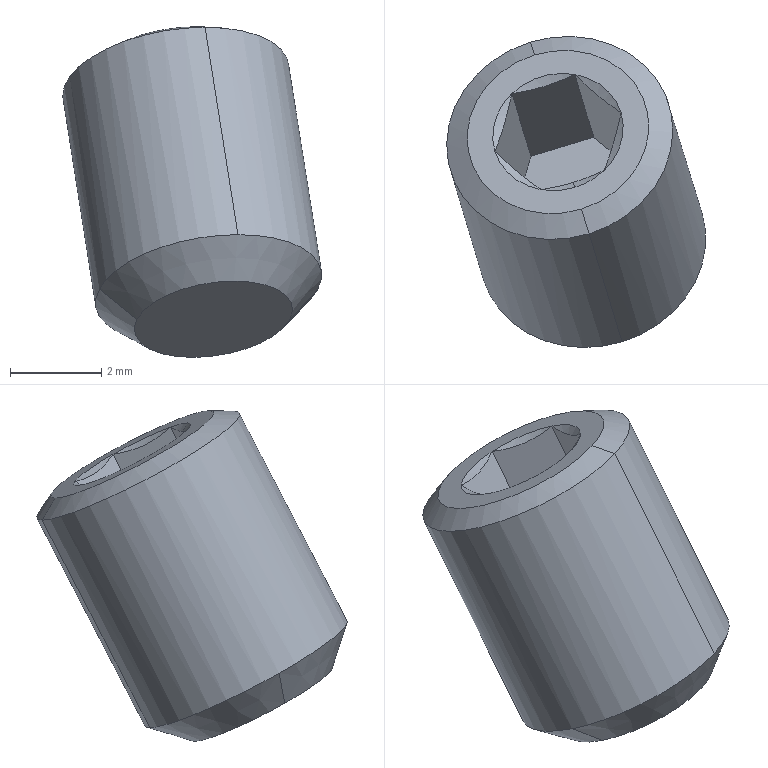Component | SolidWorks | v1ZHXTPLNY20SB1-1_v1ZHXTHeadless_pin_DIN_913_M5x8SB1-1 | 1 solid | 22 faces | box 5.67 x 6.81 x 7.24 mm | volume 100 mm3 | cone 11 | plane 9 | cylinder 2 | commonest cylinder face diameters 5 x2
STEP:
#1=COLOUR_RGB('',0.7922,0.8196,0.9333);
#2=FILL_AREA_STYLE_COLOUR('',#1);
#3=FILL_AREA_STYLE('',(#2));
#4=SURFACE_STYLE_FILL_AREA(#3);
#5=SURFACE_SIDE_STYLE('',(#4));
#6=SURFACE_STYLE_USAGE(.BOTH.,#5);
#7=PRESENTATION_STYLE_ASSIGNMENT((#6));
#8=CARTESIAN_POINT('',(6.008,-9.239,15.119));
#9=VERTEX_POINT('',#8);
#10=CARTESIAN_POINT('',(5.876,-9.279,15.119));
#11=VERTEX_POINT('',#10);
#12=CARTESIAN_POINT('',(5.942,-9.259,15.119));
#13=DIRECTION('',(-0.1392,0.4563,0.8789));
#14=DIRECTION('',(0.9565,0.2918,0.));
#15=AXIS2_PLACEMENT_3D('',#12,#13,#14);
#16=CIRCLE('',#15,0.0689);
#17=EDGE_CURVE('',#9,#11,#16,.T.);
#18=ORIENTED_EDGE('',*,*,#17,.T.);
#19=CARTESIAN_POINT('',(5.844,-9.274,15.145));
#20=VERTEX_POINT('',#19);
#21=CARTESIAN_POINT('',(5.831,-9.272,15.156));
#22=DIRECTION('',(-0.7748,0.1163,0.6215));
#23=VECTOR('',#22,39.37);
#24=LINE('',#21,#23);
#25=EDGE_CURVE('',#11,#20,#24,.T.);
#26=ORIENTED_EDGE('',*,*,#25,.T.);
#27=CARTESIAN_POINT('',(5.913,-9.163,15.098));
#28=VERTEX_POINT('',#27);
#29=CARTESIAN_POINT('',(5.938,-9.246,15.145));
#30=DIRECTION('',(-0.1392,0.4563,0.8789));
#31=DIRECTION('',(0.9565,0.2918,0.));
#32=AXIS2_PLACEMENT_3D('',#29,#30,#31);
#33=CIRCLE('',#32,0.09843);
#34=EDGE_CURVE('',#28,#20,#33,.T.);
#35=ORIENTED_EDGE('',*,*,#34,.F.);
#36=CARTESIAN_POINT('',(6.032,-9.217,15.145));
#37=VERTEX_POINT('',#36);
#38=CARTESIAN_POINT('',(5.938,-9.246,15.145));
#39=DIRECTION('',(-0.1392,0.4563,0.8789));
#40=DIRECTION('',(0.9565,0.2918,0.));
#41=AXIS2_PLACEMENT_3D('',#38,#39,#40);
#42=CIRCLE('',#41,0.09843);
#43=EDGE_CURVE('',#37,#28,#42,.T.);
#44=ORIENTED_EDGE('',*,*,#43,.F.);
#45=CARTESIAN_POINT('',(6.042,-9.208,15.156));
#46=DIRECTION('',(0.5779,0.529,0.6215));
#47=VECTOR('',#46,39.37);
#48=LINE('',#45,#47);
#49=EDGE_CURVE('',#9,#37,#48,.T.);
#50=ORIENTED_EDGE('',*,*,#49,.F.);
#51=EDGE_LOOP('',(#18,#26,#35,#44,#50));
#52=FACE_OUTER_BOUND('',#51,.T.);
#53=CARTESIAN_POINT('',(5.937,-9.24,15.156));
#54=DIRECTION('',(-0.1392,0.4563,0.8789));
#55=DIRECTION('',(0.9565,0.2918,0.));
#56=AXIS2_PLACEMENT_3D('',#53,#54,#55);
#57=CONICAL_SURFACE('',#56,0.1102,0.7854);
#58=ADVANCED_FACE('',(#52),#57,.T.);
#59=CARTESIAN_POINT('',(5.929,-9.214,15.371));
#60=VERTEX_POINT('',#59);
#61=CARTESIAN_POINT('',(5.888,-9.081,15.296));
#62=VERTEX_POINT('',#61);
#63=CARTESIAN_POINT('',(5.908,-9.148,15.334));
#64=DIRECTION('',(-0.1392,0.4563,0.8789));
#65=DIRECTION('',(0.2565,-0.8406,0.4771));
#66=AXIS2_PLACEMENT_3D('',#63,#64,#65);
#67=CIRCLE('',#66,0.07911);
#68=EDGE_CURVE('',#60,#62,#67,.T.);
#69=ORIENTED_EDGE('',*,*,#68,.F.);
#70=CARTESIAN_POINT('',(5.935,-9.235,15.371));
#71=VERTEX_POINT('',#70);
#72=CARTESIAN_POINT('',(5.929,-9.214,15.371));
#73=DIRECTION('',(0.2917,-0.9561,-0.0263));
#74=VECTOR('',#73,39.37);
#75=LINE('',#72,#74);
#76=EDGE_CURVE('',#60,#71,#75,.T.);
#77=ORIENTED_EDGE('',*,*,#76,.T.);
#78=CARTESIAN_POINT('',(5.885,-9.07,15.277));
#79=VERTEX_POINT('',#78);
#80=CARTESIAN_POINT('',(5.91,-9.153,15.324));
#81=DIRECTION('',(-0.1392,0.4563,0.8789));
#82=DIRECTION('',(0.2565,-0.8406,0.4771));
#83=AXIS2_PLACEMENT_3D('',#80,#81,#82);
#84=CIRCLE('',#83,0.09843);
#85=EDGE_CURVE('',#71,#79,#84,.T.);
#86=ORIENTED_EDGE('',*,*,#85,.T.);
#87=CARTESIAN_POINT('',(5.888,-9.081,15.296));
#88=DIRECTION('',(-0.1525,0.4999,-0.8526));
#89=VECTOR('',#88,39.37);
#90=LINE('',#87,#89);
#91=EDGE_CURVE('',#62,#79,#90,.T.);
#92=ORIENTED_EDGE('',*,*,#91,.F.);
#93=EDGE_LOOP('',(#69,#77,#86,#92));
#94=FACE_OUTER_BOUND('',#93,.T.);
#95=CARTESIAN_POINT('',(5.908,-9.148,15.334));
#96=DIRECTION('',(0.1392,-0.4563,-0.8789));
#97=DIRECTION('',(-0.2565,0.8406,-0.4771));
#98=AXIS2_PLACEMENT_3D('',#95,#96,#97);
#99=CONICAL_SURFACE('',#98,0.07911,1.047);
#100=ADVANCED_FACE('',(#94),#99,.T.);
#101=CARTESIAN_POINT('',(5.948,-9.181,15.357));
#102=VERTEX_POINT('',#101);
#103=CARTESIAN_POINT('',(5.922,-9.191,15.353));
#104=VERTEX_POINT('',#103);
#105=CARTESIAN_POINT('',(5.948,-9.181,15.357));
#106=CARTESIAN_POINT('',(5.944,-9.183,15.356));
#107=CARTESIAN_POINT('',(5.94,-9.185,15.355));
#108=CARTESIAN_POINT('',(5.931,-9.188,15.354));
#109=CARTESIAN_POINT('',(5.926,-9.19,15.353));
#110=CARTESIAN_POINT('',(5.922,-9.191,15.353));
#111=B_SPLINE_CURVE_WITH_KNOTS('',3,(#105,#106,#107,#108,#109,#110),.UNSPECIFIED.,.F.,.F.,(4,2,4),(0.003865,0.004231,0.004596),.UNSPECIFIED.);
#112=EDGE_CURVE('',#102,#104,#111,.T.);
#113=ORIENTED_EDGE('',*,*,#112,.T.);
#114=CARTESIAN_POINT('',(5.923,-9.195,15.361));
#115=VERTEX_POINT('',#114);
#116=CARTESIAN_POINT('',(5.913,-9.163,15.305));
#117=DIRECTION('',(0.1525,-0.4999,0.8526));
#118=VECTOR('',#117,39.37);
#119=LINE('',#116,#118);
#120=EDGE_CURVE('',#104,#115,#119,.T.);
#121=ORIENTED_EDGE('',*,*,#120,.T.);
#122=CARTESIAN_POINT('',(5.908,-9.148,15.334));
#123=DIRECTION('',(-0.1392,0.4563,0.8789));
#124=DIRECTION('',(0.2565,-0.8406,0.4771));
#125=AXIS2_PLACEMENT_3D('',#122,#123,#124);
#126=CIRCLE('',#125,0.05683);
#127=EDGE_CURVE('',#115,#102,#126,.T.);
#128=ORIENTED_EDGE('',*,*,#127,.T.);
#129=EDGE_LOOP('',(#113,#121,#128));
#130=FACE_OUTER_BOUND('',#129,.T.);
#131=CARTESIAN_POINT('',(0.4318,8.801,49.906));
#132=DIRECTION('',(-0.1392,0.4563,0.8789));
#133=DIRECTION('',(0.2565,-0.8406,0.4771));
#134=AXIS2_PLACEMENT_3D('',#131,#132,#133);
#135=CONICAL_SURFACE('',#134,68.191,1.047);
#136=ADVANCED_FACE('',(#130),#135,.F.);
#137=CARTESIAN_POINT('',(5.963,-9.328,15.192));
#138=VERTEX_POINT('',#137);
#139=CARTESIAN_POINT('',(5.938,-9.246,15.145));
#140=DIRECTION('',(-0.1392,0.4563,0.8789));
#141=DIRECTION('',(0.9565,0.2918,0.));
#142=AXIS2_PLACEMENT_3D('',#139,#140,#141);
#143=CIRCLE('',#142,0.09843);
#144=EDGE_CURVE('',#138,#37,#143,.T.);
#145=ORIENTED_EDGE('',*,*,#144,.T.);
#146=ORIENTED_EDGE('',*,*,#43,.T.);
#147=CARTESIAN_POINT('',(5.888,-9.08,15.258));
#148=DIRECTION('',(-0.1392,0.4563,0.8789));
#149=VECTOR('',#148,39.37);
#150=LINE('',#147,#149);
#151=EDGE_CURVE('',#28,#79,#150,.T.);
#152=ORIENTED_EDGE('',*,*,#151,.T.);
#153=ORIENTED_EDGE('',*,*,#85,.F.);
#154=CARTESIAN_POINT('',(5.938,-9.245,15.352));
#155=DIRECTION('',(-0.1392,0.4563,0.8789));
#156=VECTOR('',#155,39.37);
#157=LINE('',#154,#156);
#158=EDGE_CURVE('',#138,#71,#157,.T.);
#159=ORIENTED_EDGE('',*,*,#158,.F.);
#160=EDGE_LOOP('',(#145,#146,#152,#153,#159));
#161=FACE_OUTER_BOUND('',#160,.T.);
#162=CARTESIAN_POINT('',(5.913,-9.163,15.305));
#163=DIRECTION('',(-0.1392,0.4563,0.8789));
#164=DIRECTION('',(0.2565,-0.8406,0.4771));
#165=AXIS2_PLACEMENT_3D('',#162,#163,#164);
#166=CYLINDRICAL_SURFACE('',#165,0.09843);
#167=ADVANCED_FACE('',(#161),#166,.T.);
#168=ORIENTED_EDGE('',*,*,#151,.F.);
#169=ORIENTED_EDGE('',*,*,#34,.T.);
#170=CARTESIAN_POINT('',(5.938,-9.246,15.145));
#171=DIRECTION('',(-0.1392,0.4563,0.8789));
#172=DIRECTION('',(0.9565,0.2918,0.));
#173=AXIS2_PLACEMENT_3D('',#170,#171,#172);
#174=CIRCLE('',#173,0.09843);
#175=EDGE_CURVE('',#20,#138,#174,.T.);
#176=ORIENTED_EDGE('',*,*,#175,.T.);
#177=ORIENTED_EDGE('',*,*,#158,.T.);
#178=CARTESIAN_POINT('',(5.91,-9.153,15.324));
#179=DIRECTION('',(-0.1392,0.4563,0.8789));
#180=DIRECTION('',(0.2565,-0.8406,0.4771));
#181=AXIS2_PLACEMENT_3D('',#178,#179,#180);
#182=CIRCLE('',#181,0.09843);
#183=EDGE_CURVE('',#79,#71,#182,.T.);
#184=ORIENTED_EDGE('',*,*,#183,.F.);
#185=EDGE_LOOP('',(#168,#169,#176,#177,#184));
#186=FACE_OUTER_BOUND('',#185,.T.);
#187=CARTESIAN_POINT('',(5.913,-9.163,15.305));
#188=DIRECTION('',(-0.1392,0.4563,0.8789));
#189=DIRECTION('',(0.2565,-0.8406,0.4771));
#190=AXIS2_PLACEMENT_3D('',#187,#188,#189);
#191=CYLINDRICAL_SURFACE('',#190,0.09843);
#192=ADVANCED_FACE('',(#186),#191,.T.);
#193=CARTESIAN_POINT('',(5.963,-9.131,15.334));
#194=VERTEX_POINT('',#193);
#195=CARTESIAN_POINT('',(5.923,-9.098,15.31));
#196=VERTEX_POINT('',#195);
#197=CARTESIAN_POINT('',(5.908,-9.148,15.334));
#198=DIRECTION('',(-0.1392,0.4563,0.8789));
#199=DIRECTION('',(0.2565,-0.8406,0.4771));
#200=AXIS2_PLACEMENT_3D('',#197,#198,#199);
#201=CIRCLE('',#200,0.05683);
#202=EDGE_CURVE('',#194,#196,#201,.T.);
#203=ORIENTED_EDGE('',*,*,#202,.T.);
#204=CARTESIAN_POINT('',(5.923,-9.098,15.31));
#205=CARTESIAN_POINT('',(5.93,-9.105,15.312));
#206=CARTESIAN_POINT('',(5.937,-9.111,15.314));
#207=CARTESIAN_POINT('',(5.95,-9.122,15.322));
#208=CARTESIAN_POINT('',(5.957,-9.127,15.328));
#209=CARTESIAN_POINT('',(5.963,-9.131,15.334));
#210=B_SPLINE_CURVE_WITH_KNOTS('',3,(#204,#205,#206,#207,#208,#209),.UNSPECIFIED.,.F.,.F.,(4,2,4),(0.00000024,0.0007291,0.001458),.UNSPECIFIED.);
#211=EDGE_CURVE('',#196,#194,#210,.T.);
#212=ORIENTED_EDGE('',*,*,#211,.T.);
#213=EDGE_LOOP('',(#203,#212));
#214=FACE_OUTER_BOUND('',#213,.T.);
#215=CARTESIAN_POINT('',(0.4318,8.801,49.906));
#216=DIRECTION('',(-0.1392,0.4563,0.8789));
#217=DIRECTION('',(0.2565,-0.8406,0.4771));
#218=AXIS2_PLACEMENT_3D('',#215,#216,#217);
#219=CONICAL_SURFACE('',#218,68.191,1.047);
#220=ADVANCED_FACE('',(#214),#219,.F.);
#221=CARTESIAN_POINT('',(5.908,-9.148,15.334));
#222=DIRECTION('',(-0.1392,0.4563,0.8789));
#223=DIRECTION('',(0.2565,-0.8406,0.4771));
#224=AXIS2_PLACEMENT_3D('',#221,#222,#223);
#225=CIRCLE('',#224,0.05683);
#226=EDGE_CURVE('',#102,#194,#225,.T.);
#227=ORIENTED_EDGE('',*,*,#226,.T.);
#228=CARTESIAN_POINT('',(5.963,-9.131,15.334));
#229=CARTESIAN_POINT('',(5.961,-9.14,15.335));
#230=CARTESIAN_POINT('',(5.959,-9.149,15.338));
#231=CARTESIAN_POINT('',(5.954,-9.166,15.346));
#232=CARTESIAN_POINT('',(5.951,-9.174,15.351));
#233=CARTESIAN_POINT('',(5.948,-9.181,15.357));
#234=B_SPLINE_CURVE_WITH_KNOTS('',3,(#228,#229,#230,#231,#232,#233),.UNSPECIFIED.,.F.,.F.,(4,2,4),(0.00000024,0.0007291,0.001458),.UNSPECIFIED.);
#235=EDGE_CURVE('',#194,#102,#234,.T.);
#236=ORIENTED_EDGE('',*,*,#235,.T.);
#237=EDGE_LOOP('',(#227,#236));
#238=FACE_OUTER_BOUND('',#237,.T.);
#239=CARTESIAN_POINT('',(0.4318,8.801,49.906));
#240=DIRECTION('',(-0.1392,0.4563,0.8789));
#241=DIRECTION('',(0.2565,-0.8406,0.4771));
#242=AXIS2_PLACEMENT_3D('',#239,#240,#241);
#243=CONICAL_SURFACE('',#242,68.191,1.047);
#244=ADVANCED_FACE('',(#238),#243,.F.);
#245=ORIENTED_EDGE('',*,*,#120,.F.);
#246=CARTESIAN_POINT('',(5.894,-9.197,15.357));
#247=VERTEX_POINT('',#246);
#248=CARTESIAN_POINT('',(5.922,-9.191,15.353));
#249=CARTESIAN_POINT('',(5.912,-9.194,15.353));
#250=CARTESIAN_POINT('',(5.903,-9.196,15.355));
#251=CARTESIAN_POINT('',(5.894,-9.197,15.357));
#252=B_SPLINE_CURVE_WITH_KNOTS('',3,(#248,#249,#250,#251),.UNSPECIFIED.,.F.,.F.,(4,4),(0.004596,0.005327),.UNSPECIFIED.);
#253=EDGE_CURVE('',#104,#247,#252,.T.);
#254=ORIENTED_EDGE('',*,*,#253,.T.);
#255=CARTESIAN_POINT('',(5.908,-9.148,15.334));
#256=DIRECTION('',(-0.1392,0.4563,0.8789));
#257=DIRECTION('',(0.2565,-0.8406,0.4771));
#258=AXIS2_PLACEMENT_3D('',#255,#256,#257);
#259=CIRCLE('',#258,0.05683);
#260=EDGE_CURVE('',#247,#115,#259,.T.);
#261=ORIENTED_EDGE('',*,*,#260,.T.);
#262=EDGE_LOOP('',(#245,#254,#261));
#263=FACE_OUTER_BOUND('',#262,.T.);
#264=CARTESIAN_POINT('',(0.4318,8.801,49.906));
#265=DIRECTION('',(-0.1392,0.4563,0.8789));
#266=DIRECTION('',(0.2565,-0.8406,0.4771));
#267=AXIS2_PLACEMENT_3D('',#264,#265,#266);
#268=CONICAL_SURFACE('',#267,68.191,1.047);
#269=ADVANCED_FACE('',(#263),#268,.F.);
#270=CARTESIAN_POINT('',(5.854,-9.164,15.334));
#271=VERTEX_POINT('',#270);
#272=CARTESIAN_POINT('',(5.908,-9.148,15.334));
#273=DIRECTION('',(-0.1392,0.4563,0.8789));
#274=DIRECTION('',(0.2565,-0.8406,0.4771));
#275=AXIS2_PLACEMENT_3D('',#272,#273,#274);
#276=CIRCLE('',#275,0.05683);
#277=EDGE_CURVE('',#271,#247,#276,.T.);
#278=ORIENTED_EDGE('',*,*,#277,.T.);
#279=CARTESIAN_POINT('',(5.894,-9.197,15.357));
#280=CARTESIAN_POINT('',(5.888,-9.193,15.351));
#281=CARTESIAN_POINT('',(5.881,-9.188,15.346));
#282=CARTESIAN_POINT('',(5.868,-9.177,15.338));
#283=CARTESIAN_POINT('',(5.861,-9.171,15.335));
#284=CARTESIAN_POINT('',(5.854,-9.164,15.334));
#285=B_SPLINE_CURVE_WITH_KNOTS('',3,(#279,#280,#281,#282,#283,#284),.UNSPECIFIED.,.F.,.F.,(4,2,4),(0.00000024,0.0007291,0.001458),.UNSPECIFIED.);
#286=EDGE_CURVE('',#247,#271,#285,.T.);
#287=ORIENTED_EDGE('',*,*,#286,.T.);
#288=EDGE_LOOP('',(#278,#287));
#289=FACE_OUTER_BOUND('',#288,.T.);
#290=CARTESIAN_POINT('',(0.4318,8.801,49.906));
#291=DIRECTION('',(-0.1392,0.4563,0.8789));
#292=DIRECTION('',(0.2565,-0.8406,0.4771));
#293=AXIS2_PLACEMENT_3D('',#290,#291,#292);
#294=CONICAL_SURFACE('',#293,68.191,1.047);
#295=ADVANCED_FACE('',(#289),#294,.F.);
#296=CARTESIAN_POINT('',(5.869,-9.115,15.31));
#297=VERTEX_POINT('',#296);
#298=CARTESIAN_POINT('',(5.908,-9.148,15.334));
#299=DIRECTION('',(-0.1392,0.4563,0.8789));
#300=DIRECTION('',(0.2565,-0.8406,0.4771));
#301=AXIS2_PLACEMENT_3D('',#298,#299,#300);
#302=CIRCLE('',#301,0.05683);
#303=EDGE_CURVE('',#297,#271,#302,.T.);
#304=ORIENTED_EDGE('',*,*,#303,.T.);
#305=CARTESIAN_POINT('',(5.854,-9.164,15.334));
#306=CARTESIAN_POINT('',(5.857,-9.157,15.328));
#307=CARTESIAN_POINT('',(5.859,-9.15,15.322));
#308=CARTESIAN_POINT('',(5.864,-9.133,15.314));
#309=CARTESIAN_POINT('',(5.867,-9.124,15.312));
#310=CARTESIAN_POINT('',(5.869,-9.115,15.31));
#311=B_SPLINE_CURVE_WITH_KNOTS('',3,(#305,#306,#307,#308,#309,#310),.UNSPECIFIED.,.F.,.F.,(4,2,4),(0.00000024,0.0007291,0.001458),.UNSPECIFIED.);
#312=EDGE_CURVE('',#271,#297,#311,.T.);
#313=ORIENTED_EDGE('',*,*,#312,.T.);
#314=EDGE_LOOP('',(#304,#313));
#315=FACE_OUTER_BOUND('',#314,.T.);
#316=CARTESIAN_POINT('',(0.4318,8.801,49.906));
#317=DIRECTION('',(-0.1392,0.4563,0.8789));
#318=DIRECTION('',(0.2565,-0.8406,0.4771));
#319=AXIS2_PLACEMENT_3D('',#316,#317,#318);
#320=CONICAL_SURFACE('',#319,68.191,1.047);
#321=ADVANCED_FACE('',(#315),#320,.F.);
#322=CARTESIAN_POINT('',(5.908,-9.148,15.334));
#323=DIRECTION('',(-0.1392,0.4563,0.8789));
#324=DIRECTION('',(0.2565,-0.8406,0.4771));
#325=AXIS2_PLACEMENT_3D('',#322,#323,#324);
#326=CIRCLE('',#325,0.05683);
#327=EDGE_CURVE('',#196,#297,#326,.T.);
#328=ORIENTED_EDGE('',*,*,#327,.T.);
#329=CARTESIAN_POINT('',(5.869,-9.115,15.31));
#330=CARTESIAN_POINT('',(5.878,-9.113,15.308));
#331=CARTESIAN_POINT('',(5.887,-9.111,15.306));
#332=CARTESIAN_POINT('',(5.901,-9.107,15.306));
#333=CARTESIAN_POINT('',(5.906,-9.105,15.307));
#334=CARTESIAN_POINT('',(5.914,-9.102,15.308));
#335=CARTESIAN_POINT('',(5.919,-9.1,15.309));
#336=CARTESIAN_POINT('',(5.923,-9.098,15.31));
#337=B_SPLINE_CURVE_WITH_KNOTS('',3,(#329,#330,#331,#332,#333,#334,#335,#336),.UNSPECIFIED.,.F.,.F.,(4,2,2,4),(0.001238,0.001967,0.002332,0.002697),.UNSPECIFIED.);
#338=EDGE_CURVE('',#297,#196,#337,.T.);
#339=ORIENTED_EDGE('',*,*,#338,.T.);
#340=EDGE_LOOP('',(#328,#339));
#341=FACE_OUTER_BOUND('',#340,.T.);
#342=CARTESIAN_POINT('',(0.4318,8.801,49.906));
#343=DIRECTION('',(-0.1392,0.4563,0.8789));
#344=DIRECTION('',(0.2565,-0.8406,0.4771));
#345=AXIS2_PLACEMENT_3D('',#342,#343,#344);
#346=CONICAL_SURFACE('',#345,68.191,1.047);
#347=ADVANCED_FACE('',(#341),#346,.F.);
#348=ORIENTED_EDGE('',*,*,#76,.F.);
#349=CARTESIAN_POINT('',(5.908,-9.148,15.334));
#350=DIRECTION('',(-0.1392,0.4563,0.8789));
#351=DIRECTION('',(0.2565,-0.8406,0.4771));
#352=AXIS2_PLACEMENT_3D('',#349,#350,#351);
#353=CIRCLE('',#352,0.07911);
#354=EDGE_CURVE('',#62,#60,#353,.T.);
#355=ORIENTED_EDGE('',*,*,#354,.F.);
#356=ORIENTED_EDGE('',*,*,#91,.T.);
#357=ORIENTED_EDGE('',*,*,#183,.T.);
#358=EDGE_LOOP('',(#348,#355,#356,#357));
#359=FACE_OUTER_BOUND('',#358,.T.);
#360=CARTESIAN_POINT('',(5.908,-9.148,15.334));
#361=DIRECTION('',(0.1392,-0.4563,-0.8789));
#362=DIRECTION('',(-0.2565,0.8406,-0.4771));
#363=AXIS2_PLACEMENT_3D('',#360,#361,#362);
#364=CONICAL_SURFACE('',#363,0.07911,1.047);
#365=ADVANCED_FACE('',(#359),#364,.T.);
#366=ORIENTED_EDGE('',*,*,#354,.T.);
#367=ORIENTED_EDGE('',*,*,#68,.T.);
#368=EDGE_LOOP('',(#366,#367));
#369=FACE_OUTER_BOUND('',#368,.T.);
#370=ORIENTED_EDGE('',*,*,#226,.F.);
#371=ORIENTED_EDGE('',*,*,#127,.F.);
#372=ORIENTED_EDGE('',*,*,#260,.F.);
#373=ORIENTED_EDGE('',*,*,#277,.F.);
#374=ORIENTED_EDGE('',*,*,#303,.F.);
#375=ORIENTED_EDGE('',*,*,#327,.F.);
#376=ORIENTED_EDGE('',*,*,#202,.F.);
#377=EDGE_LOOP('',(#370,#371,#372,#373,#374,#375,#376));
#378=FACE_BOUND('',#377,.T.);
#379=CARTESIAN_POINT('',(5.929,-9.214,15.371));
#380=DIRECTION('',(-0.1392,0.4563,0.8789));
#381=DIRECTION('',(0.2565,-0.8406,0.4771));
#382=AXIS2_PLACEMENT_3D('',#379,#380,#381);
#383=PLANE('',#382);
#384=ADVANCED_FACE('',(#369,#378),#383,.T.);
#385=CARTESIAN_POINT('',(5.939,-9.152,15.206));
#386=VERTEX_POINT('',#385);
#387=CARTESIAN_POINT('',(5.939,-9.152,15.206));
#388=DIRECTION('',(-0.1392,0.4563,0.8789));
#389=VECTOR('',#388,39.37);
#390=LINE('',#387,#389);
#391=EDGE_CURVE('',#386,#196,#390,.T.);
#392=ORIENTED_EDGE('',*,*,#391,.F.);
#393=CARTESIAN_POINT('',(5.979,-9.185,15.23));
#394=VERTEX_POINT('',#393);
#395=CARTESIAN_POINT('',(5.939,-9.152,15.206));
#396=DIRECTION('',(0.7004,-0.5821,0.4131));
#397=VECTOR('',#396,39.37);
#398=LINE('',#395,#397);
#399=EDGE_CURVE('',#386,#394,#398,.T.);
#400=ORIENTED_EDGE('',*,*,#399,.T.);
#401=CARTESIAN_POINT('',(5.979,-9.185,15.23));
#402=DIRECTION('',(-0.1392,0.4563,0.8789));
#403=VECTOR('',#402,39.37);
#404=LINE('',#401,#403);
#405=EDGE_CURVE('',#394,#194,#404,.T.);
#406=ORIENTED_EDGE('',*,*,#405,.T.);
#407=ORIENTED_EDGE('',*,*,#211,.F.);
#408=EDGE_LOOP('',(#392,#400,#406,#407));
#409=FACE_OUTER_BOUND('',#408,.T.);
#410=CARTESIAN_POINT('',(5.939,-9.152,15.206));
#411=DIRECTION('',(-0.7001,-0.673,0.2385));
#412=DIRECTION('',(-0.7004,0.5821,-0.4131));
#413=AXIS2_PLACEMENT_3D('',#410,#411,#412);
#414=PLANE('',#413);
#415=ADVANCED_FACE('',(#409),#414,.T.);
#416=ORIENTED_EDGE('',*,*,#405,.F.);
#417=CARTESIAN_POINT('',(5.965,-9.235,15.253));
#418=VERTEX_POINT('',#417);
#419=CARTESIAN_POINT('',(5.979,-9.185,15.23));
#420=DIRECTION('',(-0.2561,-0.8739,0.4131));
#421=VECTOR('',#420,39.37);
#422=LINE('',#419,#421);
#423=EDGE_CURVE('',#394,#418,#422,.T.);
#424=ORIENTED_EDGE('',*,*,#423,.T.);
#425=CARTESIAN_POINT('',(5.965,-9.235,15.253));
#426=DIRECTION('',(-0.1392,0.4563,0.8789));
#427=VECTOR('',#426,39.37);
#428=LINE('',#425,#427);
#429=EDGE_CURVE('',#418,#102,#428,.T.);
#430=ORIENTED_EDGE('',*,*,#429,.T.);
#431=ORIENTED_EDGE('',*,*,#235,.F.);
#432=EDGE_LOOP('',(#416,#424,#430,#431));
#433=FACE_OUTER_BOUND('',#432,.T.);
#434=CARTESIAN_POINT('',(5.979,-9.185,15.23));
#435=DIRECTION('',(-0.9566,0.1676,-0.2385));
#436=DIRECTION('',(0.2561,0.8739,-0.4131));
#437=AXIS2_PLACEMENT_3D('',#434,#435,#436);
#438=PLANE('',#437);
#439=ADVANCED_FACE('',(#433),#438,.T.);
#440=ORIENTED_EDGE('',*,*,#429,.F.);
#441=CARTESIAN_POINT('',(5.91,-9.251,15.253));
#442=VERTEX_POINT('',#441);
#443=CARTESIAN_POINT('',(5.965,-9.235,15.253));
#444=DIRECTION('',(-0.9565,-0.2918,-0.));
#445=VECTOR('',#444,39.37);
#446=LINE('',#443,#445);
#447=EDGE_CURVE('',#418,#442,#446,.T.);
#448=ORIENTED_EDGE('',*,*,#447,.T.);
#449=CARTESIAN_POINT('',(5.91,-9.251,15.253));
#450=DIRECTION('',(-0.1392,0.4563,0.8789));
#451=VECTOR('',#450,39.37);
#452=LINE('',#449,#451);
#453=EDGE_CURVE('',#442,#247,#452,.T.);
#454=ORIENTED_EDGE('',*,*,#453,.T.);
#455=ORIENTED_EDGE('',*,*,#253,.F.);
#456=ORIENTED_EDGE('',*,*,#112,.F.);
#457=EDGE_LOOP('',(#440,#448,#454,#455,#456));
#458=FACE_OUTER_BOUND('',#457,.T.);
#459=CARTESIAN_POINT('',(5.965,-9.235,15.253));
#460=DIRECTION('',(-0.2565,0.8406,-0.4771));
#461=DIRECTION('',(0.9565,0.2918,0.));
#462=AXIS2_PLACEMENT_3D('',#459,#460,#461);
#463=PLANE('',#462);
#464=ADVANCED_FACE('',(#458),#463,.T.);
#465=ORIENTED_EDGE('',*,*,#453,.F.);
#466=CARTESIAN_POINT('',(5.87,-9.218,15.23));
#467=VERTEX_POINT('',#466);
#468=CARTESIAN_POINT('',(5.91,-9.251,15.253));
#469=DIRECTION('',(-0.7004,0.5821,-0.4131));
#470=VECTOR('',#469,39.37);
#471=LINE('',#468,#470);
#472=EDGE_CURVE('',#442,#467,#471,.T.);
#473=ORIENTED_EDGE('',*,*,#472,.T.);
#474=CARTESIAN_POINT('',(5.87,-9.218,15.23));
#475=DIRECTION('',(-0.1392,0.4563,0.8789));
#476=VECTOR('',#475,39.37);
#477=LINE('',#474,#476);
#478=EDGE_CURVE('',#467,#271,#477,.T.);
#479=ORIENTED_EDGE('',*,*,#478,.T.);
#480=ORIENTED_EDGE('',*,*,#286,.F.);
#481=EDGE_LOOP('',(#465,#473,#479,#480));
#482=FACE_OUTER_BOUND('',#481,.T.);
#483=CARTESIAN_POINT('',(5.91,-9.251,15.253));
#484=DIRECTION('',(0.7001,0.673,-0.2385));
#485=DIRECTION('',(0.7004,-0.5821,0.4131));
#486=AXIS2_PLACEMENT_3D('',#483,#484,#485);
#487=PLANE('',#486);
#488=ADVANCED_FACE('',(#482),#487,.T.);
#489=ORIENTED_EDGE('',*,*,#478,.F.);
#490=CARTESIAN_POINT('',(5.885,-9.168,15.206));
#491=VERTEX_POINT('',#490);
#492=CARTESIAN_POINT('',(5.87,-9.218,15.23));
#493=DIRECTION('',(0.2561,0.8739,-0.4131));
#494=VECTOR('',#493,39.37);
#495=LINE('',#492,#494);
#496=EDGE_CURVE('',#467,#491,#495,.T.);
#497=ORIENTED_EDGE('',*,*,#496,.T.);
#498=CARTESIAN_POINT('',(5.885,-9.168,15.206));
#499=DIRECTION('',(-0.1392,0.4563,0.8789));
#500=VECTOR('',#499,39.37);
#501=LINE('',#498,#500);
#502=EDGE_CURVE('',#491,#297,#501,.T.);
#503=ORIENTED_EDGE('',*,*,#502,.T.);
#504=ORIENTED_EDGE('',*,*,#312,.F.);
#505=EDGE_LOOP('',(#489,#497,#503,#504));
#506=FACE_OUTER_BOUND('',#505,.T.);
#507=CARTESIAN_POINT('',(5.87,-9.218,15.23));
#508=DIRECTION('',(0.9566,-0.1676,0.2385));
#509=DIRECTION('',(-0.2561,-0.8739,0.4131));
#510=AXIS2_PLACEMENT_3D('',#507,#508,#509);
#511=PLANE('',#510);
#512=ADVANCED_FACE('',(#506),#511,.T.);
#513=ORIENTED_EDGE('',*,*,#502,.F.);
#514=CARTESIAN_POINT('',(5.885,-9.168,15.206));
#515=DIRECTION('',(0.9565,0.2918,0.));
#516=VECTOR('',#515,39.37);
#517=LINE('',#514,#516);
#518=EDGE_CURVE('',#491,#386,#517,.T.);
#519=ORIENTED_EDGE('',*,*,#518,.T.);
#520=ORIENTED_EDGE('',*,*,#391,.T.);
#521=ORIENTED_EDGE('',*,*,#338,.F.);
#522=EDGE_LOOP('',(#513,#519,#520,#521));
#523=FACE_OUTER_BOUND('',#522,.T.);
#524=CARTESIAN_POINT('',(5.885,-9.168,15.206));
#525=DIRECTION('',(0.2565,-0.8406,0.4771));
#526=DIRECTION('',(-0.9565,-0.2918,-0.));
#527=AXIS2_PLACEMENT_3D('',#524,#525,#526);
#528=PLANE('',#527);
#529=ADVANCED_FACE('',(#523),#528,.T.);
#530=ORIENTED_EDGE('',*,*,#399,.F.);
#531=ORIENTED_EDGE('',*,*,#518,.F.);
#532=ORIENTED_EDGE('',*,*,#496,.F.);
#533=ORIENTED_EDGE('',*,*,#472,.F.);
#534=ORIENTED_EDGE('',*,*,#447,.F.);
#535=ORIENTED_EDGE('',*,*,#423,.F.);
#536=EDGE_LOOP('',(#530,#531,#532,#533,#534,#535));
#537=FACE_OUTER_BOUND('',#536,.T.);
#538=CARTESIAN_POINT('',(5.925,-9.202,15.23));
#539=DIRECTION('',(0.1392,-0.4563,-0.8789));
#540=DIRECTION('',(-0.9565,-0.2918,-0.));
#541=AXIS2_PLACEMENT_3D('',#538,#539,#540);
#542=PLANE('',#541);
#543=ADVANCED_FACE('',(#537),#542,.F.);
#544=ORIENTED_EDGE('',*,*,#17,.F.);
#545=CARTESIAN_POINT('',(5.942,-9.259,15.119));
#546=DIRECTION('',(-0.1392,0.4563,0.8789));
#547=DIRECTION('',(0.9565,0.2918,0.));
#548=AXIS2_PLACEMENT_3D('',#545,#546,#547);
#549=CIRCLE('',#548,0.0689);
#550=EDGE_CURVE('',#11,#9,#549,.T.);
#551=ORIENTED_EDGE('',*,*,#550,.F.);
#552=EDGE_LOOP('',(#544,#551));
#553=FACE_OUTER_BOUND('',#552,.T.);
#554=CARTESIAN_POINT('',(5.925,-9.201,15.086));
#555=DIRECTION('',(0.1392,-0.4563,-0.8789));
#556=DIRECTION('',(-0.9565,-0.2918,-0.));
#557=AXIS2_PLACEMENT_3D('',#554,#555,#556);
#558=PLANE('',#557);
#559=ADVANCED_FACE('',(#553),#558,.T.);
#560=ORIENTED_EDGE('',*,*,#25,.F.);
#561=ORIENTED_EDGE('',*,*,#550,.T.);
#562=ORIENTED_EDGE('',*,*,#49,.T.);
#563=ORIENTED_EDGE('',*,*,#144,.F.);
#564=ORIENTED_EDGE('',*,*,#175,.F.);
#565=EDGE_LOOP('',(#560,#561,#562,#563,#564));
#566=FACE_OUTER_BOUND('',#565,.T.);
#567=CARTESIAN_POINT('',(5.937,-9.24,15.156));
#568=DIRECTION('',(-0.1392,0.4563,0.8789));
#569=DIRECTION('',(0.9565,0.2918,0.));
#570=AXIS2_PLACEMENT_3D('',#567,#568,#569);
#571=CONICAL_SURFACE('',#570,0.1102,0.7854);
#572=ADVANCED_FACE('',(#566),#571,.T.);
#573=CLOSED_SHELL('',(#58,#100,#136,#167,#192,#220,#244,#269,#295,#321,#347,#365,#384,#415,#439,#464,#488,#512,#529,#543,#559,#572));
#574=MANIFOLD_SOLID_BREP('',#573);
#575=STYLED_ITEM('',(#7),#574);
#576=(LENGTH_UNIT()NAMED_UNIT(*)SI_UNIT($,.METRE.));
#577=LENGTH_MEASURE_WITH_UNIT(LENGTH_MEASURE(0.0254),#576);
#578=DIMENSIONAL_EXPONENTS(1.,0.,0.,0.,0.,0.,0.);
#579=(CONVERSION_BASED_UNIT('',#577)LENGTH_UNIT()NAMED_UNIT(#578));
#580=UNCERTAINTY_MEASURE_WITH_UNIT(LENGTH_MEASURE(0.00001),#579,'','');
#581=(NAMED_UNIT(*)PLANE_ANGLE_UNIT()SI_UNIT($,.RADIAN.));
#582=(NAMED_UNIT(*)SI_UNIT($,.STERADIAN.)SOLID_ANGLE_UNIT());
#583=(GEOMETRIC_REPRESENTATION_CONTEXT(3)GLOBAL_UNCERTAINTY_ASSIGNED_CONTEXT((#580))GLOBAL_UNIT_ASSIGNED_CONTEXT((#579,#581,#582))REPRESENTATION_CONTEXT('',''));
#584=MECHANICAL_DESIGN_GEOMETRIC_PRESENTATION_REPRESENTATION('',(#575),#583);
#585=PRESENTATION_LAYER_ASSIGNMENT('','',(#575));
#586=CARTESIAN_POINT('',(0.,0.,0.));
#587=DIRECTION('',(0.,0.,1.));
#588=DIRECTION('',(1.,0.,0.));
#589=AXIS2_PLACEMENT_3D('',#586,#587,#588);
#590=(LENGTH_UNIT()NAMED_UNIT(*)SI_UNIT($,.METRE.));
#591=LENGTH_MEASURE_WITH_UNIT(LENGTH_MEASURE(0.0254),#590);
#592=DIMENSIONAL_EXPONENTS(1.,0.,0.,0.,0.,0.,0.);
#593=(CONVERSION_BASED_UNIT('',#591)LENGTH_UNIT()NAMED_UNIT(#592));
#594=UNCERTAINTY_MEASURE_WITH_UNIT(LENGTH_MEASURE(0.00001),#593,'','');
#595=(NAMED_UNIT(*)PLANE_ANGLE_UNIT()SI_UNIT($,.RADIAN.));
#596=(NAMED_UNIT(*)SI_UNIT($,.STERADIAN.)SOLID_ANGLE_UNIT());
#597=(GEOMETRIC_REPRESENTATION_CONTEXT(3)GLOBAL_UNCERTAINTY_ASSIGNED_CONTEXT((#594))GLOBAL_UNIT_ASSIGNED_CONTEXT((#593,#595,#596))REPRESENTATION_CONTEXT('',''));
#598=ADVANCED_BREP_SHAPE_REPRESENTATION('',(#574,#589),#597);